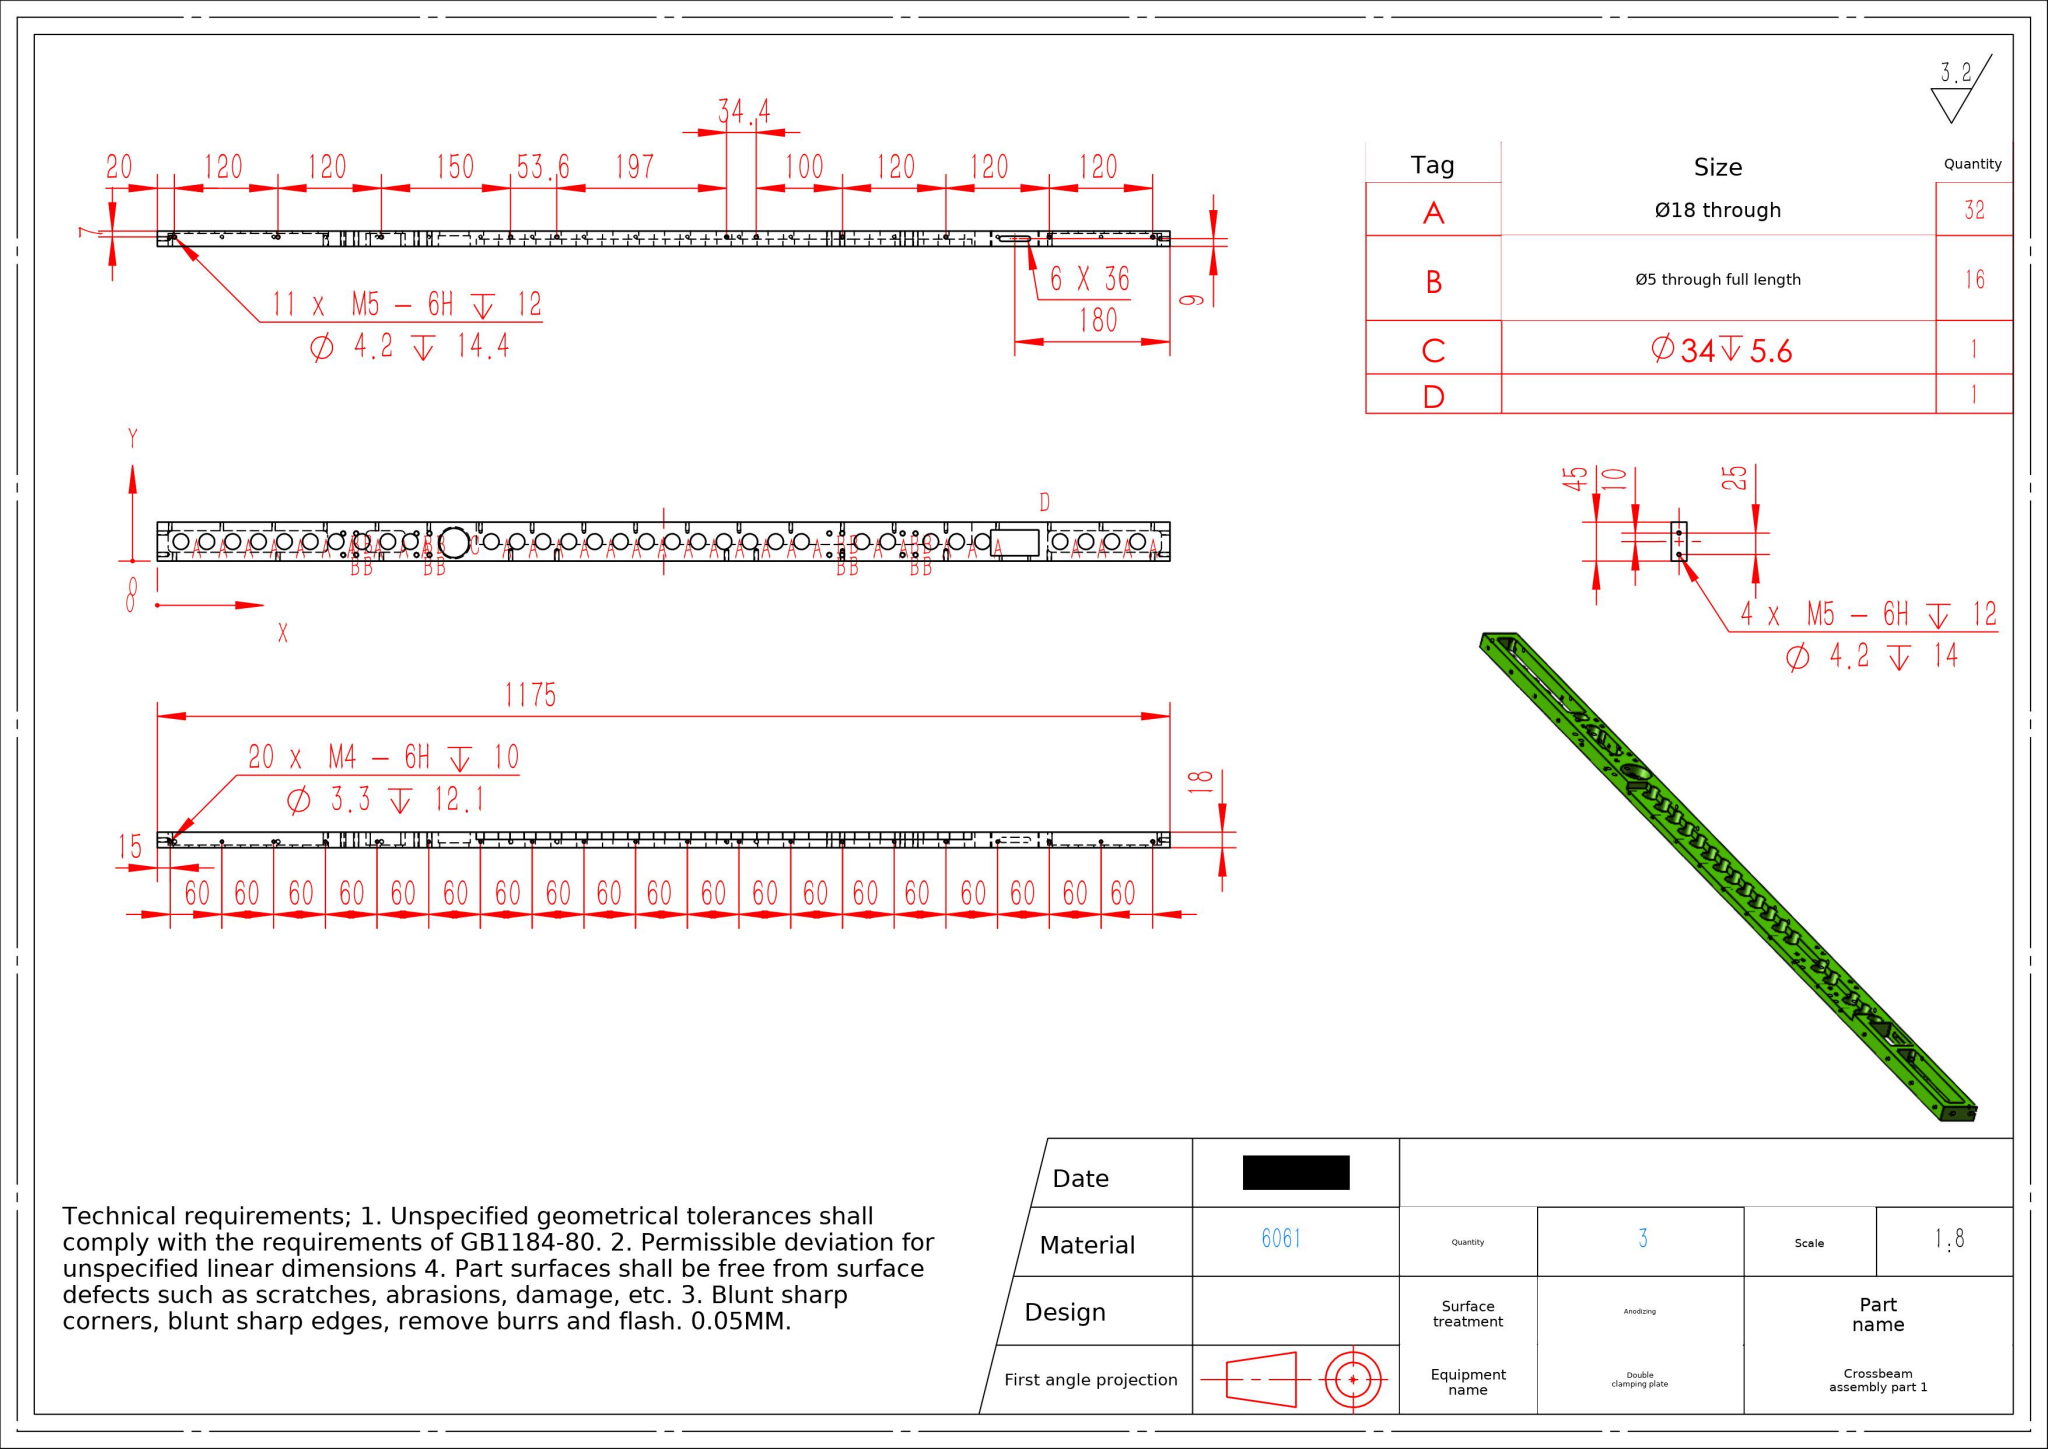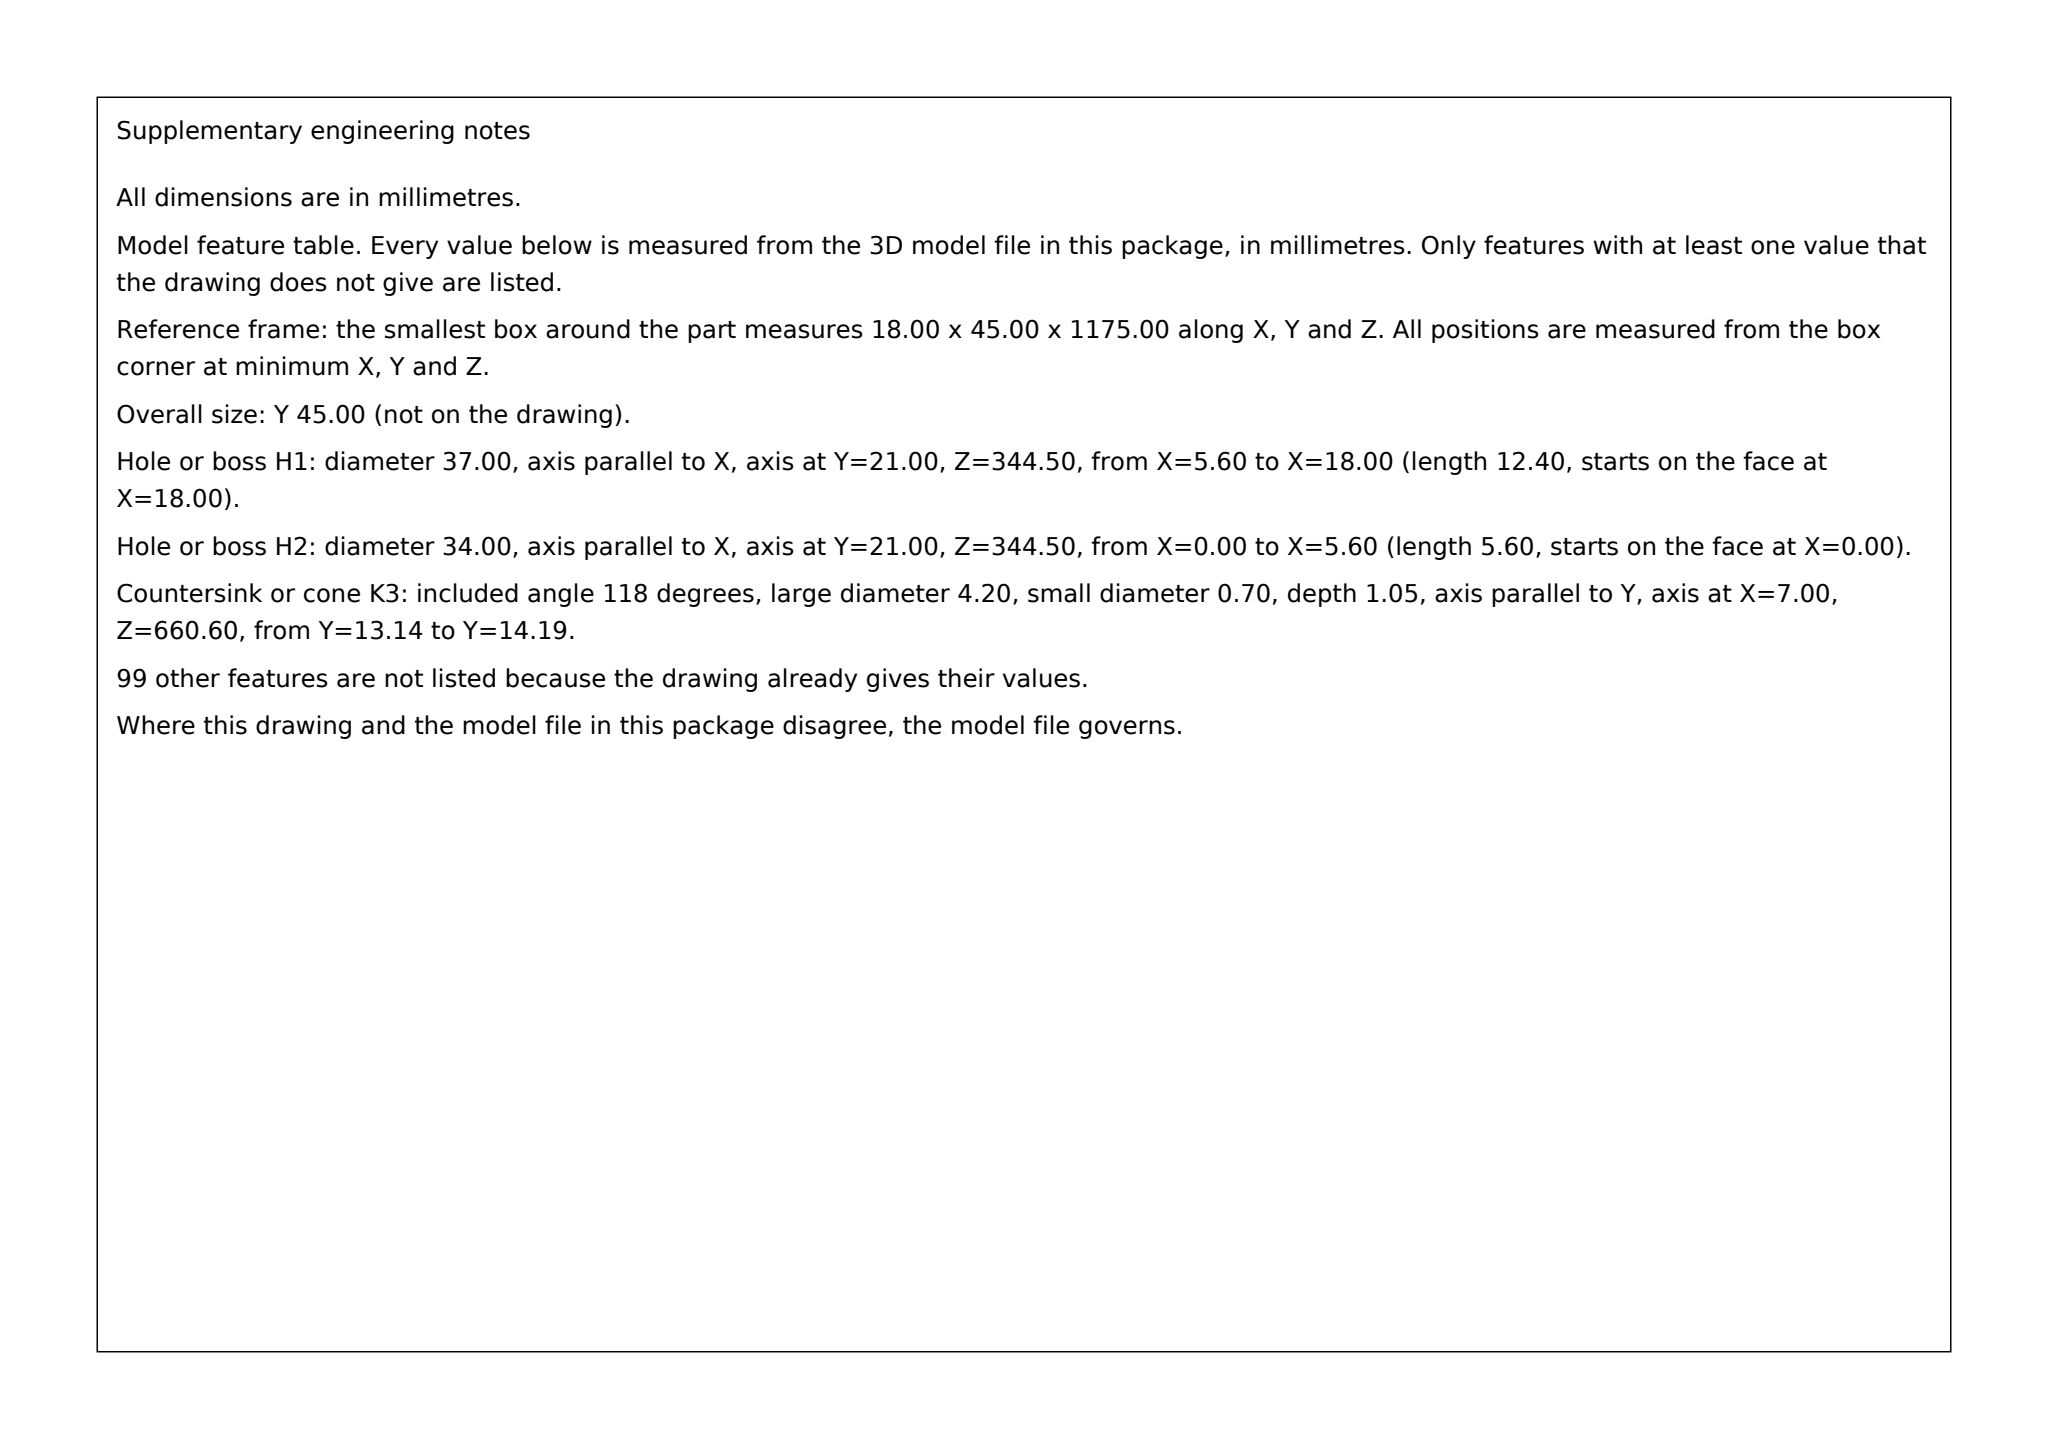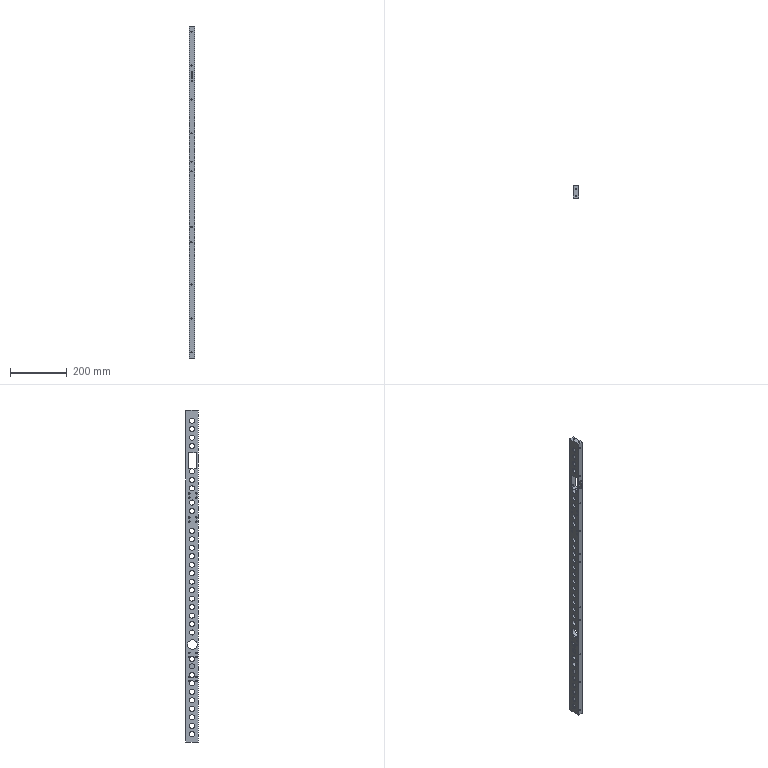Part | SolidWorks | mm | material 6061 | 1 solid | 278 faces | box 18 x 45 x 1175 mm | volume 555437 mm3 | cylinder 191 | plane 50 | cone 37 | commonest cylinder face diameters 18 x64 3.3 x40 4.2 x32 5 x32 10 x12 2 x4 6 x3 34 x2